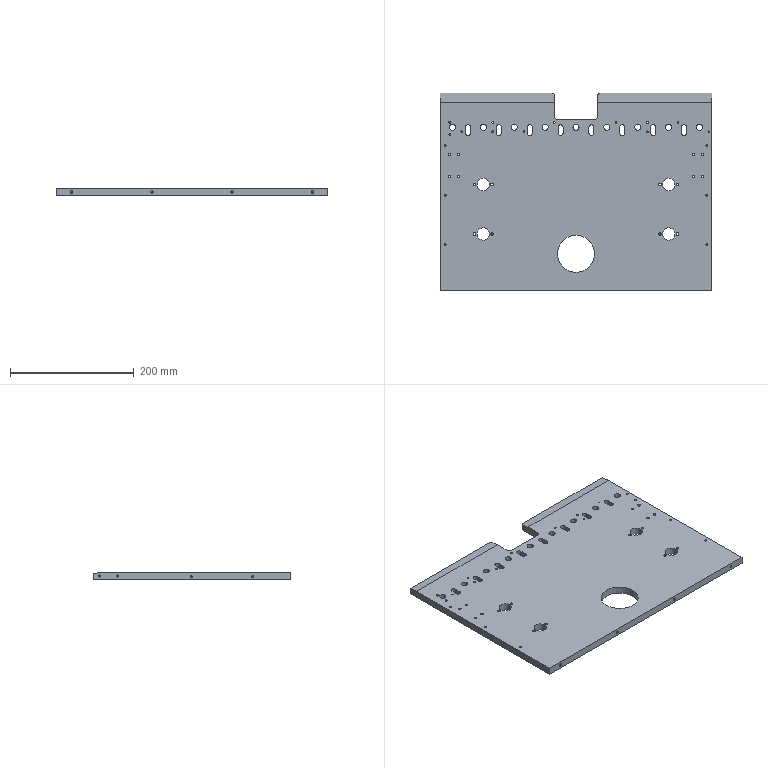Component | SolidWorks | 002MaterialPickingModuleB-1_J-001-1 | 1 solid | 206 faces | volume 1567064 mm3 | cylinder 146 | plane 32 | cone 28 | commonest cylinder face diameters 4.2 x40 3.3 x36 10 x22 2.5 x16 8 x16 20 x8 3 x4 60 x2 | material 45